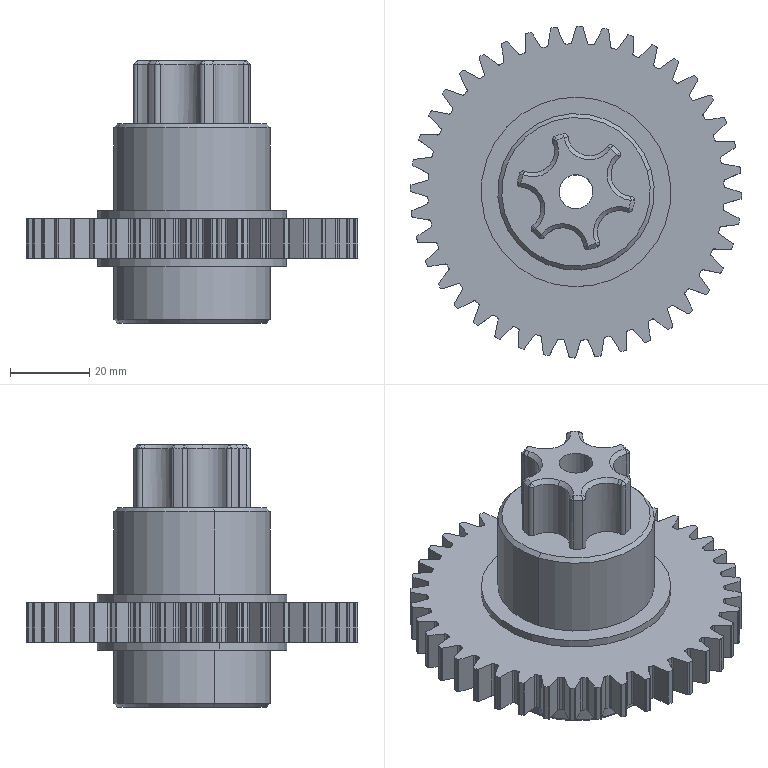Component | SolidWorks | DriveDevice-1_LargeGear-1 | 1 solid | 445 faces | volume 100439 mm3 | cylinder 316 | plane 94 | cone 35 | commonest cylinder face diameters 1 x98 0.6 x96 84 x41 75 x40 2 x16 11 x9 30 x6 39.6 x4